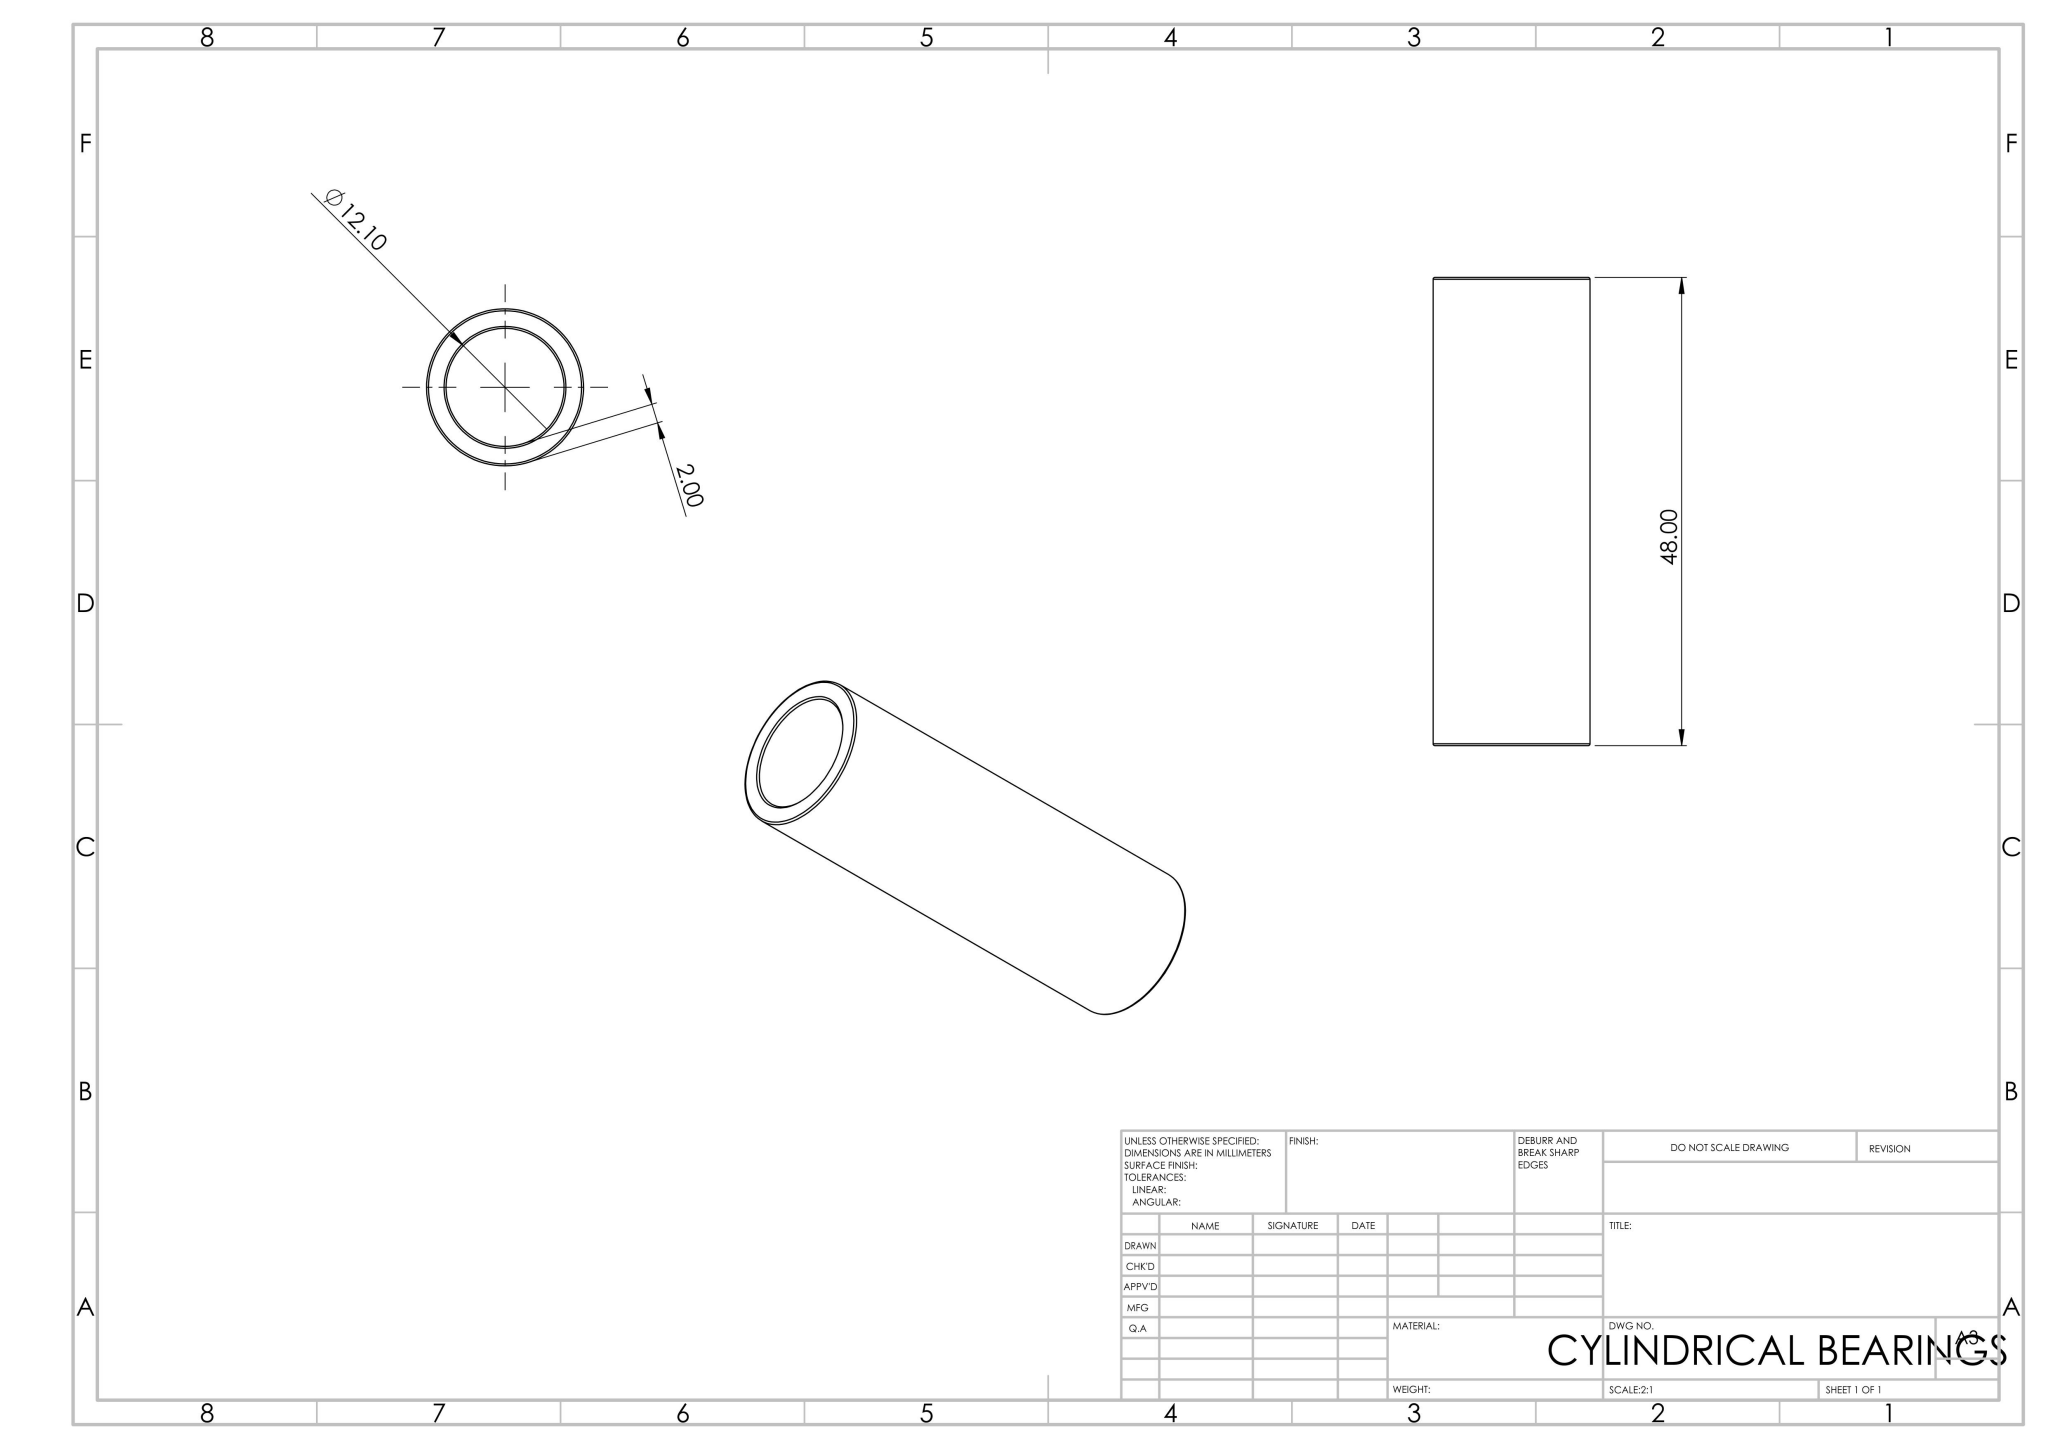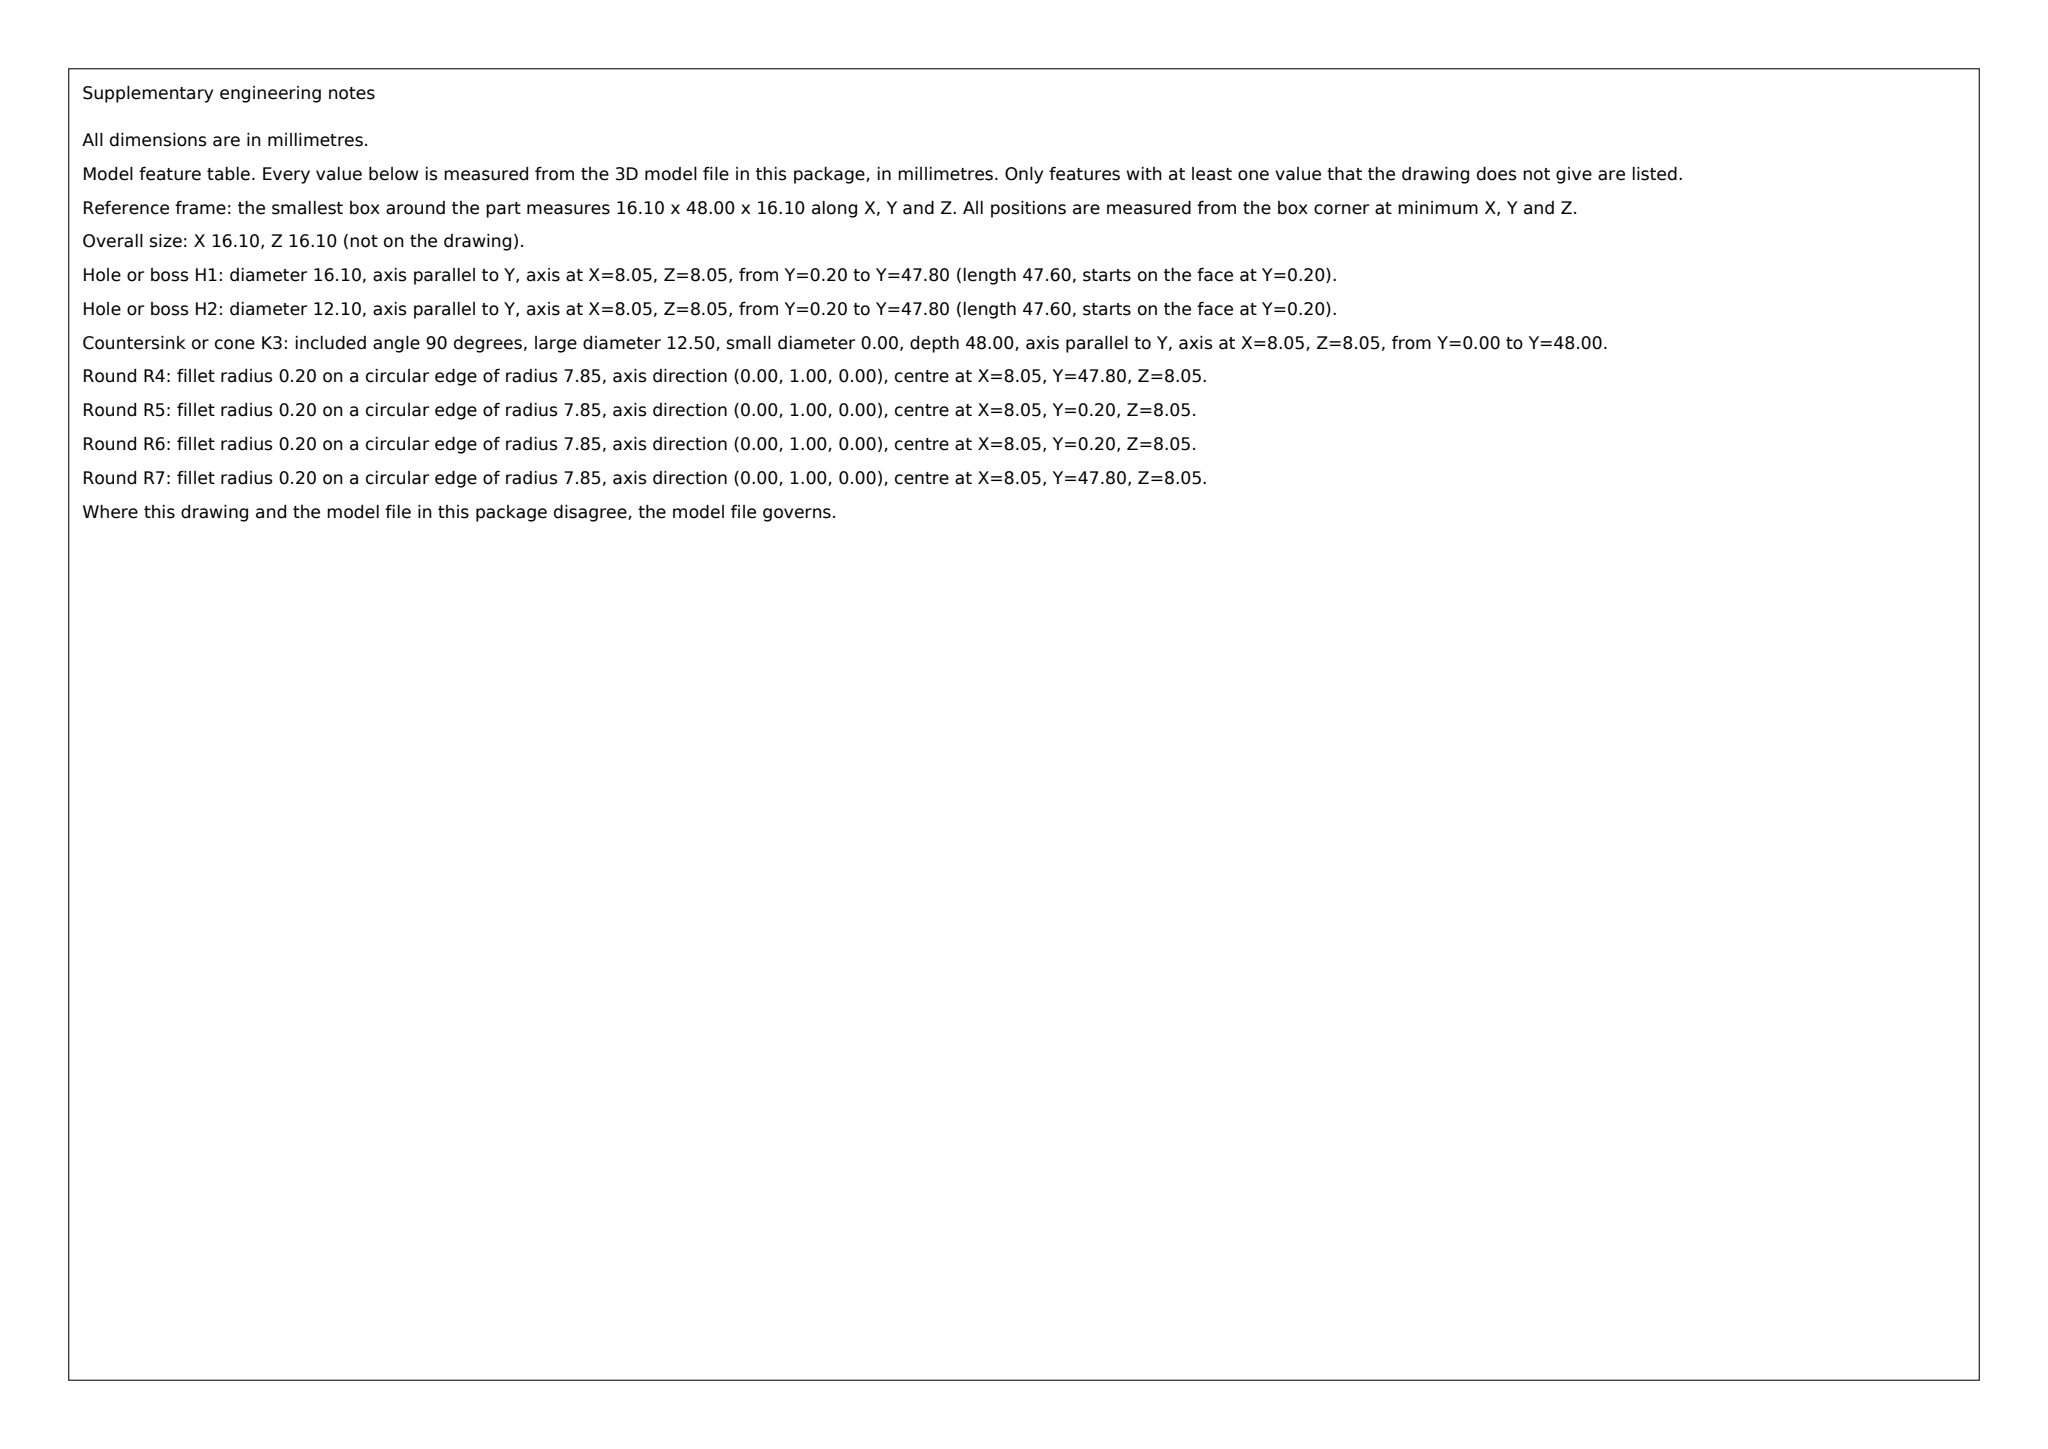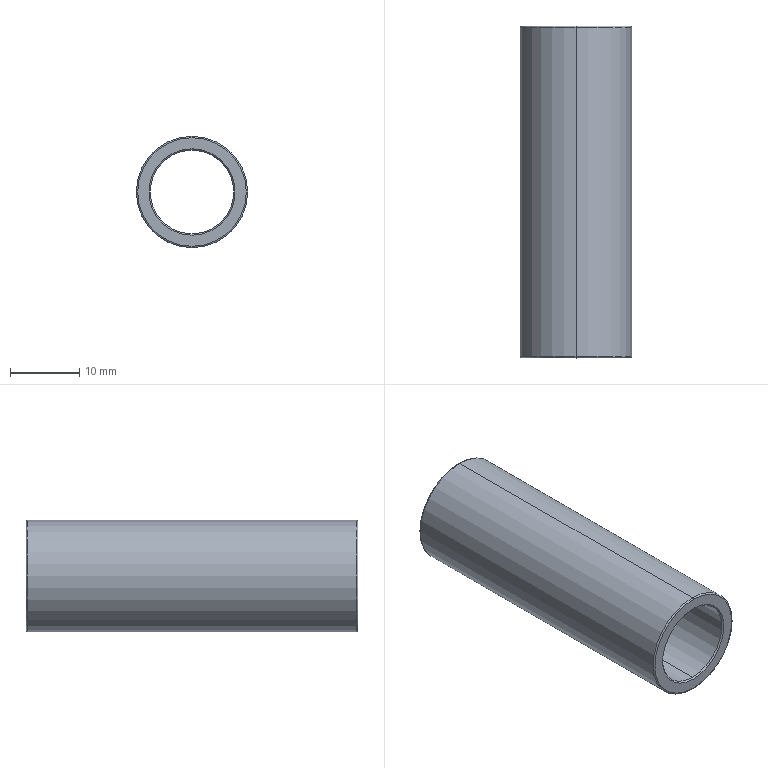Part | SolidWorks | mm | 1 solid | 14 faces | box 16.1 x 48 x 16.1 mm | volume 4250 mm3 | torus 4 | cone 4 | cylinder 4 | plane 2 | commonest cylinder face diameters 12.1 x2 16.1 x2
build123d program:
from build123d import *

# Parameters (mm, degrees)
SKETCH1_R           = 8.05
SKETCH1_R_2         = 6.05
BOSS_EXTRUDE1_DEPTH = 48
CHAMFER1_SIZE       = 0.2
FILLET1_R           = 0.2


with BuildPart() as part:
    # Sketch1 → Boss-Extrude1 (new body)
    with BuildSketch(Plane(origin=(0, 0, 0), x_dir=(1, 0, 0), z_dir=(0, 1, 0))):
        with Locations(Location((0, 0, 0), (0, 0, 270))):
            Circle(SKETCH1_R)
        with Locations(Location((0, 0, 0), (0, 0, 270))):
            Circle(SKETCH1_R_2, mode=Mode.SUBTRACT)
    extrude(amount=BOSS_EXTRUDE1_DEPTH)

    # Chamfer1
    chamfer1_edges = [part.edges().sort_by_distance(p)[0] for p in [
        (0, 0, -6.05),
        (0, 48, -6.05),
    ]]
    chamfer(chamfer1_edges, length=CHAMFER1_SIZE)

    # Fillet1
    fillet1_edges = [part.edges().sort_by_distance(p)[0] for p in [
        (0, 0, -8.05),
        (0, 48, -8.05),
    ]]
    fillet(fillet1_edges, radius=FILLET1_R)


solid = part.part
STEP:
#1=CARTESIAN_POINT('',(0.,47.8,-8.05));
#2=VERTEX_POINT('',#1);
#3=CARTESIAN_POINT('',(0.,47.8,8.05));
#4=VERTEX_POINT('',#3);
#5=CARTESIAN_POINT('',(0.,47.8,0.));
#6=DIRECTION('',(0.,-1.,0.));
#7=DIRECTION('',(0.,0.,1.));
#8=AXIS2_PLACEMENT_3D('',#5,#6,#7);
#9=CIRCLE('',#8,8.05);
#10=EDGE_CURVE('',#2,#4,#9,.T.);
#11=ORIENTED_EDGE('',*,*,#10,.F.);
#12=CARTESIAN_POINT('',(0.,48.,-7.85));
#13=VERTEX_POINT('',#12);
#14=CARTESIAN_POINT('',(0.,47.8,-7.85));
#15=DIRECTION('',(1.,0.,0.));
#16=DIRECTION('',(0.,0.,-1.));
#17=AXIS2_PLACEMENT_3D('',#14,#15,#16);
#18=CIRCLE('',#17,0.2);
#19=EDGE_CURVE('',#2,#13,#18,.T.);
#20=ORIENTED_EDGE('',*,*,#19,.T.);
#21=CARTESIAN_POINT('',(0.,48.,7.85));
#22=VERTEX_POINT('',#21);
#23=CARTESIAN_POINT('',(0.,48.,0.));
#24=DIRECTION('',(0.,1.,0.));
#25=DIRECTION('',(0.,0.,1.));
#26=AXIS2_PLACEMENT_3D('',#23,#24,#25);
#27=CIRCLE('',#26,7.85);
#28=EDGE_CURVE('',#22,#13,#27,.T.);
#29=ORIENTED_EDGE('',*,*,#28,.F.);
#30=CARTESIAN_POINT('',(0.,47.8,7.85));
#31=DIRECTION('',(-1.,0.,0.));
#32=DIRECTION('',(0.,0.,1.));
#33=AXIS2_PLACEMENT_3D('',#30,#31,#32);
#34=CIRCLE('',#33,0.2);
#35=EDGE_CURVE('',#4,#22,#34,.T.);
#36=ORIENTED_EDGE('',*,*,#35,.F.);
#37=EDGE_LOOP('',(#11,#20,#29,#36));
#38=FACE_OUTER_BOUND('',#37,.T.);
#39=CARTESIAN_POINT('',(0.,47.8,0.));
#40=DIRECTION('',(0.,1.,0.));
#41=DIRECTION('',(0.,0.,1.));
#42=AXIS2_PLACEMENT_3D('',#39,#40,#41);
#43=TOROIDAL_SURFACE('',#42,7.85,0.2);
#44=ADVANCED_FACE('',(#38),#43,.T.);
#45=CARTESIAN_POINT('',(0.,0.,-7.85));
#46=VERTEX_POINT('',#45);
#47=CARTESIAN_POINT('',(0.,0.,7.85));
#48=VERTEX_POINT('',#47);
#49=CARTESIAN_POINT('',(0.,0.,0.));
#50=DIRECTION('',(0.,-1.,0.));
#51=DIRECTION('',(0.,0.,1.));
#52=AXIS2_PLACEMENT_3D('',#49,#50,#51);
#53=CIRCLE('',#52,7.85);
#54=EDGE_CURVE('',#46,#48,#53,.T.);
#55=ORIENTED_EDGE('',*,*,#54,.F.);
#56=CARTESIAN_POINT('',(0.,0.2,-8.05));
#57=VERTEX_POINT('',#56);
#58=CARTESIAN_POINT('',(0.,0.2,-7.85));
#59=DIRECTION('',(1.,0.,0.));
#60=DIRECTION('',(0.,0.,-1.));
#61=AXIS2_PLACEMENT_3D('',#58,#59,#60);
#62=CIRCLE('',#61,0.2);
#63=EDGE_CURVE('',#46,#57,#62,.T.);
#64=ORIENTED_EDGE('',*,*,#63,.T.);
#65=CARTESIAN_POINT('',(0.,0.2,8.05));
#66=VERTEX_POINT('',#65);
#67=CARTESIAN_POINT('',(0.,0.2,0.));
#68=DIRECTION('',(0.,1.,0.));
#69=DIRECTION('',(0.,0.,1.));
#70=AXIS2_PLACEMENT_3D('',#67,#68,#69);
#71=CIRCLE('',#70,8.05);
#72=EDGE_CURVE('',#66,#57,#71,.T.);
#73=ORIENTED_EDGE('',*,*,#72,.F.);
#74=CARTESIAN_POINT('',(0.,0.2,7.85));
#75=DIRECTION('',(-1.,0.,0.));
#76=DIRECTION('',(0.,0.,1.));
#77=AXIS2_PLACEMENT_3D('',#74,#75,#76);
#78=CIRCLE('',#77,0.2);
#79=EDGE_CURVE('',#48,#66,#78,.T.);
#80=ORIENTED_EDGE('',*,*,#79,.F.);
#81=EDGE_LOOP('',(#55,#64,#73,#80));
#82=FACE_OUTER_BOUND('',#81,.T.);
#83=CARTESIAN_POINT('',(0.,0.2,0.));
#84=DIRECTION('',(0.,1.,0.));
#85=DIRECTION('',(0.,0.,1.));
#86=AXIS2_PLACEMENT_3D('',#83,#84,#85);
#87=TOROIDAL_SURFACE('',#86,7.85,0.2);
#88=ADVANCED_FACE('',(#82),#87,.T.);
#89=CARTESIAN_POINT('',(0.,47.8,-6.05));
#90=VERTEX_POINT('',#89);
#91=CARTESIAN_POINT('',(0.,47.8,6.05));
#92=VERTEX_POINT('',#91);
#93=CARTESIAN_POINT('',(0.,47.8,0.));
#94=DIRECTION('',(0.,1.,0.));
#95=DIRECTION('',(0.,0.,1.));
#96=AXIS2_PLACEMENT_3D('',#93,#94,#95);
#97=CIRCLE('',#96,6.05);
#98=EDGE_CURVE('',#90,#92,#97,.T.);
#99=ORIENTED_EDGE('',*,*,#98,.F.);
#100=CARTESIAN_POINT('',(0.,48.,-6.25));
#101=VERTEX_POINT('',#100);
#102=CARTESIAN_POINT('',(0.,47.8,-6.05));
#103=DIRECTION('',(0.,0.7071,-0.7071));
#104=VECTOR('',#103,1000.);
#105=LINE('',#102,#104);
#106=EDGE_CURVE('',#90,#101,#105,.T.);
#107=ORIENTED_EDGE('',*,*,#106,.T.);
#108=CARTESIAN_POINT('',(0.,48.,6.25));
#109=VERTEX_POINT('',#108);
#110=CARTESIAN_POINT('',(0.,48.,0.));
#111=DIRECTION('',(0.,-1.,0.));
#112=DIRECTION('',(0.,0.,1.));
#113=AXIS2_PLACEMENT_3D('',#110,#111,#112);
#114=CIRCLE('',#113,6.25);
#115=EDGE_CURVE('',#109,#101,#114,.T.);
#116=ORIENTED_EDGE('',*,*,#115,.F.);
#117=CARTESIAN_POINT('',(0.,47.8,6.05));
#118=DIRECTION('',(0.,0.7071,0.7071));
#119=VECTOR('',#118,1000.);
#120=LINE('',#117,#119);
#121=EDGE_CURVE('',#92,#109,#120,.T.);
#122=ORIENTED_EDGE('',*,*,#121,.F.);
#123=EDGE_LOOP('',(#99,#107,#116,#122));
#124=FACE_OUTER_BOUND('',#123,.T.);
#125=CARTESIAN_POINT('',(0.,47.8,0.));
#126=DIRECTION('',(0.,1.,0.));
#127=DIRECTION('',(0.,0.,1.));
#128=AXIS2_PLACEMENT_3D('',#125,#126,#127);
#129=CONICAL_SURFACE('',#128,6.05,0.7854);
#130=ADVANCED_FACE('',(#124),#129,.F.);
#131=CARTESIAN_POINT('',(0.,0.2,6.05));
#132=VERTEX_POINT('',#131);
#133=CARTESIAN_POINT('',(0.,0.2,-6.05));
#134=VERTEX_POINT('',#133);
#135=CARTESIAN_POINT('',(0.,0.2,0.));
#136=DIRECTION('',(0.,-1.,0.));
#137=DIRECTION('',(0.,0.,1.));
#138=AXIS2_PLACEMENT_3D('',#135,#136,#137);
#139=CIRCLE('',#138,6.05);
#140=EDGE_CURVE('',#132,#134,#139,.T.);
#141=ORIENTED_EDGE('',*,*,#140,.F.);
#142=CARTESIAN_POINT('',(0.,0.,6.25));
#143=VERTEX_POINT('',#142);
#144=CARTESIAN_POINT('',(0.,0.,6.25));
#145=DIRECTION('',(0.,-0.7071,0.7071));
#146=VECTOR('',#145,1000.);
#147=LINE('',#144,#146);
#148=EDGE_CURVE('',#132,#143,#147,.T.);
#149=ORIENTED_EDGE('',*,*,#148,.T.);
#150=CARTESIAN_POINT('',(0.,0.,-6.25));
#151=VERTEX_POINT('',#150);
#152=CARTESIAN_POINT('',(0.,0.,0.));
#153=DIRECTION('',(0.,1.,0.));
#154=DIRECTION('',(0.,0.,1.));
#155=AXIS2_PLACEMENT_3D('',#152,#153,#154);
#156=CIRCLE('',#155,6.25);
#157=EDGE_CURVE('',#151,#143,#156,.T.);
#158=ORIENTED_EDGE('',*,*,#157,.F.);
#159=CARTESIAN_POINT('',(0.,0.,-6.25));
#160=DIRECTION('',(0.,-0.7071,-0.7071));
#161=VECTOR('',#160,1000.);
#162=LINE('',#159,#161);
#163=EDGE_CURVE('',#134,#151,#162,.T.);
#164=ORIENTED_EDGE('',*,*,#163,.F.);
#165=EDGE_LOOP('',(#141,#149,#158,#164));
#166=FACE_OUTER_BOUND('',#165,.T.);
#167=CARTESIAN_POINT('',(0.,0.,0.));
#168=DIRECTION('',(0.,-1.,0.));
#169=DIRECTION('',(0.,0.,-1.));
#170=AXIS2_PLACEMENT_3D('',#167,#168,#169);
#171=CONICAL_SURFACE('',#170,6.25,0.7854);
#172=ADVANCED_FACE('',(#166),#171,.F.);
#173=ORIENTED_EDGE('',*,*,#98,.T.);
#174=CARTESIAN_POINT('',(0.,48.,6.05));
#175=DIRECTION('',(0.,-1.,0.));
#176=VECTOR('',#175,1000.);
#177=LINE('',#174,#176);
#178=EDGE_CURVE('',#92,#132,#177,.T.);
#179=ORIENTED_EDGE('',*,*,#178,.T.);
#180=ORIENTED_EDGE('',*,*,#140,.T.);
#181=CARTESIAN_POINT('',(0.,48.,-6.05));
#182=DIRECTION('',(0.,-1.,0.));
#183=VECTOR('',#182,1000.);
#184=LINE('',#181,#183);
#185=EDGE_CURVE('',#90,#134,#184,.T.);
#186=ORIENTED_EDGE('',*,*,#185,.F.);
#187=EDGE_LOOP('',(#173,#179,#180,#186));
#188=FACE_OUTER_BOUND('',#187,.T.);
#189=CARTESIAN_POINT('',(0.,48.,0.));
#190=DIRECTION('',(0.,-1.,0.));
#191=DIRECTION('',(0.,0.,-1.));
#192=AXIS2_PLACEMENT_3D('',#189,#190,#191);
#193=CYLINDRICAL_SURFACE('',#192,6.05);
#194=ADVANCED_FACE('',(#188),#193,.F.);
#195=ORIENTED_EDGE('',*,*,#10,.T.);
#196=CARTESIAN_POINT('',(0.,48.,8.05));
#197=DIRECTION('',(0.,-1.,0.));
#198=VECTOR('',#197,1000.);
#199=LINE('',#196,#198);
#200=EDGE_CURVE('',#4,#66,#199,.T.);
#201=ORIENTED_EDGE('',*,*,#200,.T.);
#202=ORIENTED_EDGE('',*,*,#72,.T.);
#203=CARTESIAN_POINT('',(0.,48.,-8.05));
#204=DIRECTION('',(0.,-1.,0.));
#205=VECTOR('',#204,1000.);
#206=LINE('',#203,#205);
#207=EDGE_CURVE('',#2,#57,#206,.T.);
#208=ORIENTED_EDGE('',*,*,#207,.F.);
#209=EDGE_LOOP('',(#195,#201,#202,#208));
#210=FACE_OUTER_BOUND('',#209,.T.);
#211=CARTESIAN_POINT('',(0.,48.,0.));
#212=DIRECTION('',(0.,-1.,0.));
#213=DIRECTION('',(0.,0.,-1.));
#214=AXIS2_PLACEMENT_3D('',#211,#212,#213);
#215=CYLINDRICAL_SURFACE('',#214,8.05);
#216=ADVANCED_FACE('',(#210),#215,.T.);
#217=ORIENTED_EDGE('',*,*,#28,.T.);
#218=CARTESIAN_POINT('',(0.,48.,0.));
#219=DIRECTION('',(0.,1.,0.));
#220=DIRECTION('',(0.,0.,1.));
#221=AXIS2_PLACEMENT_3D('',#218,#219,#220);
#222=CIRCLE('',#221,7.85);
#223=EDGE_CURVE('',#13,#22,#222,.T.);
#224=ORIENTED_EDGE('',*,*,#223,.T.);
#225=EDGE_LOOP('',(#217,#224));
#226=FACE_OUTER_BOUND('',#225,.T.);
#227=ORIENTED_EDGE('',*,*,#115,.T.);
#228=CARTESIAN_POINT('',(0.,48.,0.));
#229=DIRECTION('',(0.,-1.,0.));
#230=DIRECTION('',(0.,0.,1.));
#231=AXIS2_PLACEMENT_3D('',#228,#229,#230);
#232=CIRCLE('',#231,6.25);
#233=EDGE_CURVE('',#101,#109,#232,.T.);
#234=ORIENTED_EDGE('',*,*,#233,.T.);
#235=EDGE_LOOP('',(#227,#234));
#236=FACE_BOUND('',#235,.T.);
#237=CARTESIAN_POINT('',(0.,48.,0.));
#238=DIRECTION('',(0.,1.,0.));
#239=DIRECTION('',(0.,0.,1.));
#240=AXIS2_PLACEMENT_3D('',#237,#238,#239);
#241=PLANE('',#240);
#242=ADVANCED_FACE('',(#226,#236),#241,.T.);
#243=CARTESIAN_POINT('',(0.,0.,0.));
#244=DIRECTION('',(0.,-1.,0.));
#245=DIRECTION('',(0.,0.,1.));
#246=AXIS2_PLACEMENT_3D('',#243,#244,#245);
#247=CIRCLE('',#246,7.85);
#248=EDGE_CURVE('',#48,#46,#247,.T.);
#249=ORIENTED_EDGE('',*,*,#248,.T.);
#250=ORIENTED_EDGE('',*,*,#54,.T.);
#251=EDGE_LOOP('',(#249,#250));
#252=FACE_OUTER_BOUND('',#251,.T.);
#253=ORIENTED_EDGE('',*,*,#157,.T.);
#254=CARTESIAN_POINT('',(0.,0.,0.));
#255=DIRECTION('',(0.,1.,0.));
#256=DIRECTION('',(0.,0.,1.));
#257=AXIS2_PLACEMENT_3D('',#254,#255,#256);
#258=CIRCLE('',#257,6.25);
#259=EDGE_CURVE('',#143,#151,#258,.T.);
#260=ORIENTED_EDGE('',*,*,#259,.T.);
#261=EDGE_LOOP('',(#253,#260));
#262=FACE_BOUND('',#261,.T.);
#263=CARTESIAN_POINT('',(0.,0.,0.));
#264=DIRECTION('',(0.,1.,0.));
#265=DIRECTION('',(0.,0.,1.));
#266=AXIS2_PLACEMENT_3D('',#263,#264,#265);
#267=PLANE('',#266);
#268=ADVANCED_FACE('',(#252,#262),#267,.F.);
#269=ORIENTED_EDGE('',*,*,#200,.F.);
#270=CARTESIAN_POINT('',(0.,47.8,0.));
#271=DIRECTION('',(0.,-1.,0.));
#272=DIRECTION('',(0.,0.,1.));
#273=AXIS2_PLACEMENT_3D('',#270,#271,#272);
#274=CIRCLE('',#273,8.05);
#275=EDGE_CURVE('',#4,#2,#274,.T.);
#276=ORIENTED_EDGE('',*,*,#275,.T.);
#277=ORIENTED_EDGE('',*,*,#207,.T.);
#278=CARTESIAN_POINT('',(0.,0.2,0.));
#279=DIRECTION('',(0.,1.,0.));
#280=DIRECTION('',(0.,0.,1.));
#281=AXIS2_PLACEMENT_3D('',#278,#279,#280);
#282=CIRCLE('',#281,8.05);
#283=EDGE_CURVE('',#57,#66,#282,.T.);
#284=ORIENTED_EDGE('',*,*,#283,.T.);
#285=EDGE_LOOP('',(#269,#276,#277,#284));
#286=FACE_OUTER_BOUND('',#285,.T.);
#287=CARTESIAN_POINT('',(0.,48.,0.));
#288=DIRECTION('',(0.,-1.,0.));
#289=DIRECTION('',(0.,0.,-1.));
#290=AXIS2_PLACEMENT_3D('',#287,#288,#289);
#291=CYLINDRICAL_SURFACE('',#290,8.05);
#292=ADVANCED_FACE('',(#286),#291,.T.);
#293=ORIENTED_EDGE('',*,*,#178,.F.);
#294=CARTESIAN_POINT('',(0.,47.8,0.));
#295=DIRECTION('',(0.,1.,0.));
#296=DIRECTION('',(0.,0.,1.));
#297=AXIS2_PLACEMENT_3D('',#294,#295,#296);
#298=CIRCLE('',#297,6.05);
#299=EDGE_CURVE('',#92,#90,#298,.T.);
#300=ORIENTED_EDGE('',*,*,#299,.T.);
#301=ORIENTED_EDGE('',*,*,#185,.T.);
#302=CARTESIAN_POINT('',(0.,0.2,0.));
#303=DIRECTION('',(0.,-1.,0.));
#304=DIRECTION('',(0.,0.,1.));
#305=AXIS2_PLACEMENT_3D('',#302,#303,#304);
#306=CIRCLE('',#305,6.05);
#307=EDGE_CURVE('',#134,#132,#306,.T.);
#308=ORIENTED_EDGE('',*,*,#307,.T.);
#309=EDGE_LOOP('',(#293,#300,#301,#308));
#310=FACE_OUTER_BOUND('',#309,.T.);
#311=CARTESIAN_POINT('',(0.,48.,0.));
#312=DIRECTION('',(0.,-1.,0.));
#313=DIRECTION('',(0.,0.,-1.));
#314=AXIS2_PLACEMENT_3D('',#311,#312,#313);
#315=CYLINDRICAL_SURFACE('',#314,6.05);
#316=ADVANCED_FACE('',(#310),#315,.F.);
#317=ORIENTED_EDGE('',*,*,#148,.F.);
#318=ORIENTED_EDGE('',*,*,#307,.F.);
#319=ORIENTED_EDGE('',*,*,#163,.T.);
#320=ORIENTED_EDGE('',*,*,#259,.F.);
#321=EDGE_LOOP('',(#317,#318,#319,#320));
#322=FACE_OUTER_BOUND('',#321,.T.);
#323=CARTESIAN_POINT('',(0.,0.,0.));
#324=DIRECTION('',(0.,-1.,0.));
#325=DIRECTION('',(0.,0.,-1.));
#326=AXIS2_PLACEMENT_3D('',#323,#324,#325);
#327=CONICAL_SURFACE('',#326,6.25,0.7854);
#328=ADVANCED_FACE('',(#322),#327,.F.);
#329=ORIENTED_EDGE('',*,*,#106,.F.);
#330=ORIENTED_EDGE('',*,*,#299,.F.);
#331=ORIENTED_EDGE('',*,*,#121,.T.);
#332=ORIENTED_EDGE('',*,*,#233,.F.);
#333=EDGE_LOOP('',(#329,#330,#331,#332));
#334=FACE_OUTER_BOUND('',#333,.T.);
#335=CARTESIAN_POINT('',(0.,47.8,0.));
#336=DIRECTION('',(0.,1.,0.));
#337=DIRECTION('',(0.,0.,1.));
#338=AXIS2_PLACEMENT_3D('',#335,#336,#337);
#339=CONICAL_SURFACE('',#338,6.05,0.7854);
#340=ADVANCED_FACE('',(#334),#339,.F.);
#341=ORIENTED_EDGE('',*,*,#63,.F.);
#342=ORIENTED_EDGE('',*,*,#248,.F.);
#343=ORIENTED_EDGE('',*,*,#79,.T.);
#344=ORIENTED_EDGE('',*,*,#283,.F.);
#345=EDGE_LOOP('',(#341,#342,#343,#344));
#346=FACE_OUTER_BOUND('',#345,.T.);
#347=CARTESIAN_POINT('',(0.,0.2,0.));
#348=DIRECTION('',(0.,1.,0.));
#349=DIRECTION('',(0.,0.,1.));
#350=AXIS2_PLACEMENT_3D('',#347,#348,#349);
#351=TOROIDAL_SURFACE('',#350,7.85,0.2);
#352=ADVANCED_FACE('',(#346),#351,.T.);
#353=ORIENTED_EDGE('',*,*,#19,.F.);
#354=ORIENTED_EDGE('',*,*,#275,.F.);
#355=ORIENTED_EDGE('',*,*,#35,.T.);
#356=ORIENTED_EDGE('',*,*,#223,.F.);
#357=EDGE_LOOP('',(#353,#354,#355,#356));
#358=FACE_OUTER_BOUND('',#357,.T.);
#359=CARTESIAN_POINT('',(0.,47.8,0.));
#360=DIRECTION('',(0.,1.,0.));
#361=DIRECTION('',(0.,0.,1.));
#362=AXIS2_PLACEMENT_3D('',#359,#360,#361);
#363=TOROIDAL_SURFACE('',#362,7.85,0.2);
#364=ADVANCED_FACE('',(#358),#363,.T.);
#365=CLOSED_SHELL('',(#44,#88,#130,#172,#194,#216,#242,#268,#292,#316,#328,#340,#352,#364));
#366=MANIFOLD_SOLID_BREP('',#365);
#367=CARTESIAN_POINT('',(0.,0.,0.));
#368=DIRECTION('',(0.,0.,1.));
#369=DIRECTION('',(1.,0.,0.));
#370=AXIS2_PLACEMENT_3D('',#367,#368,#369);
#371=(LENGTH_UNIT()NAMED_UNIT(*)SI_UNIT(.MILLI.,.METRE.));
#372=UNCERTAINTY_MEASURE_WITH_UNIT(LENGTH_MEASURE(0.00001),#371,'','');
#373=(NAMED_UNIT(*)PLANE_ANGLE_UNIT()SI_UNIT($,.RADIAN.));
#374=(NAMED_UNIT(*)SI_UNIT($,.STERADIAN.)SOLID_ANGLE_UNIT());
#375=(GEOMETRIC_REPRESENTATION_CONTEXT(3)GLOBAL_UNCERTAINTY_ASSIGNED_CONTEXT((#372))GLOBAL_UNIT_ASSIGNED_CONTEXT((#371,#373,#374))REPRESENTATION_CONTEXT('',''));
#376=ADVANCED_BREP_SHAPE_REPRESENTATION('',(#366,#370),#375);